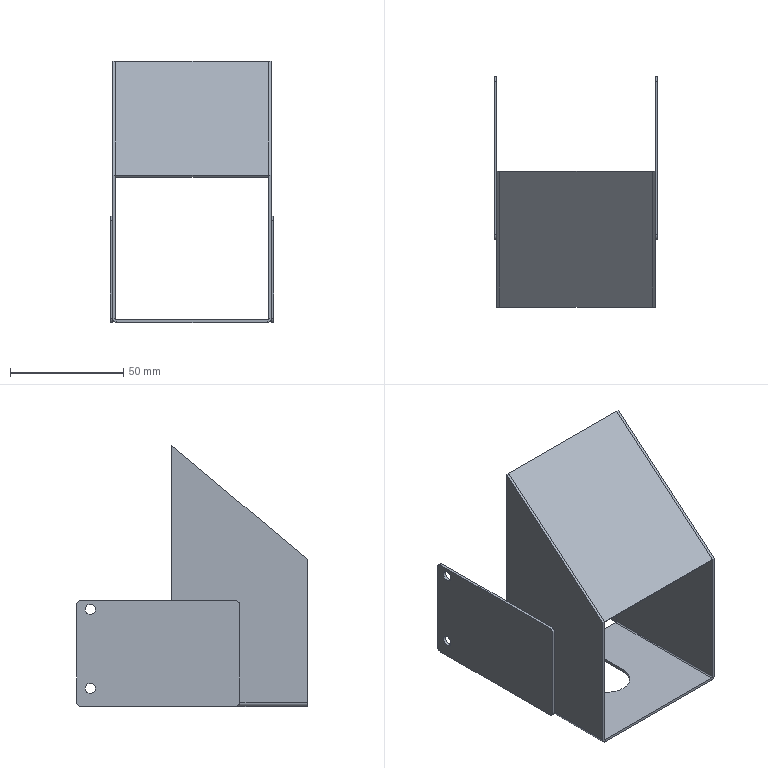Component | SolidWorks | BAssemblyInnerBagFunnel-1_InnerBagFunnel2-1 | 4 solids | 61 faces | volume 31299 mm3 | plane 39 | cylinder 22 | commonest cylinder face diameters 4.5 x8 4 x8 20 x2 3.4 x2 1 x2